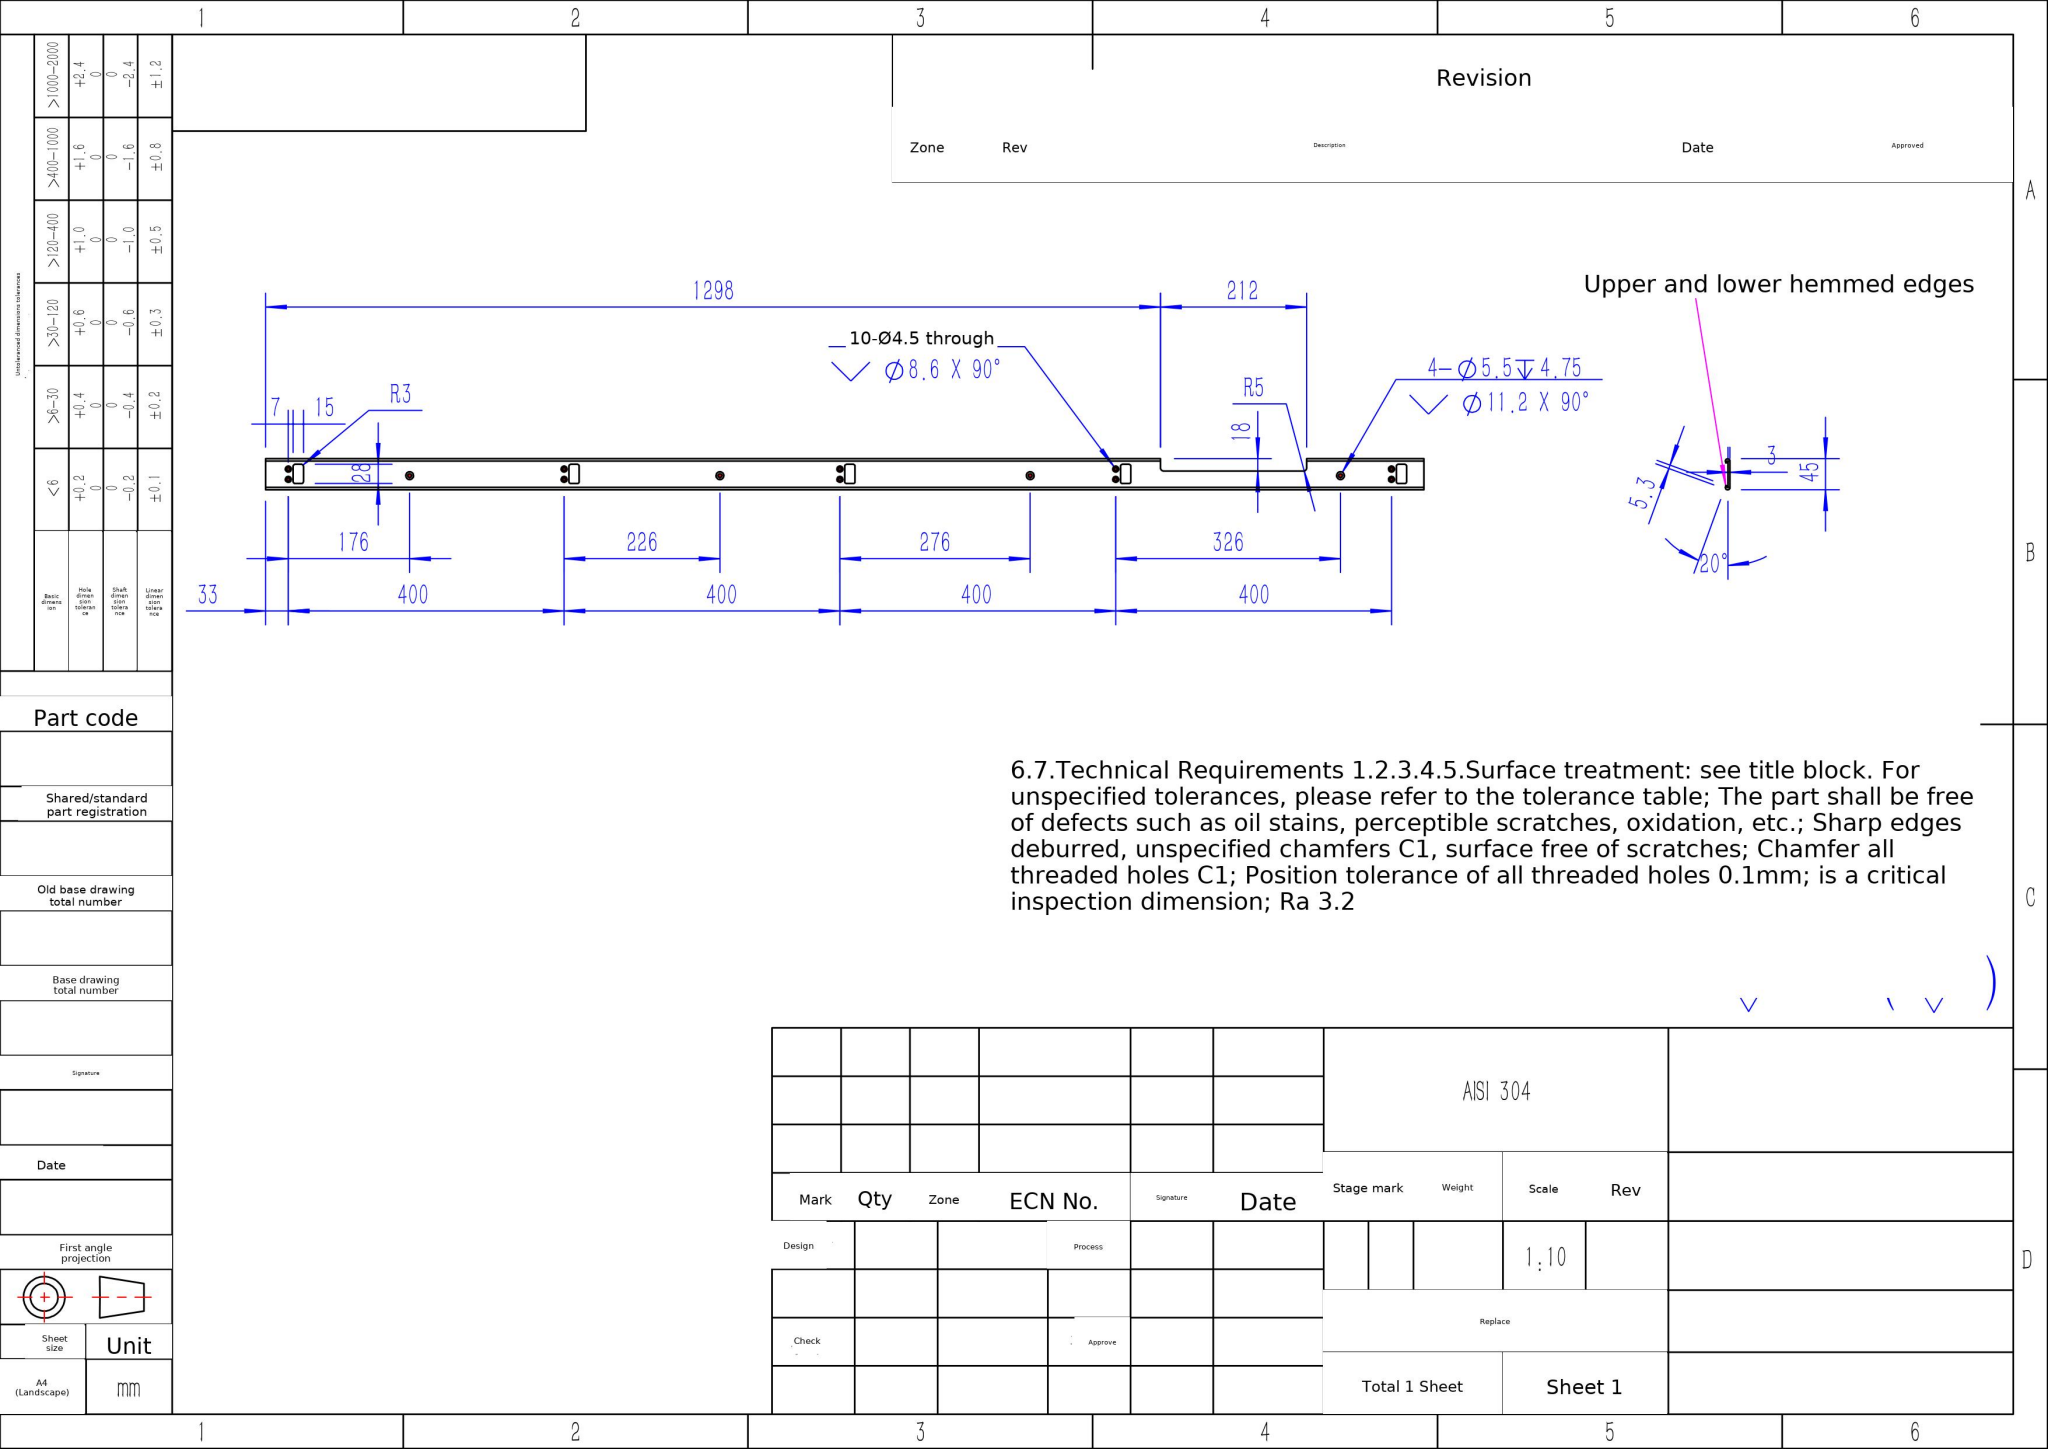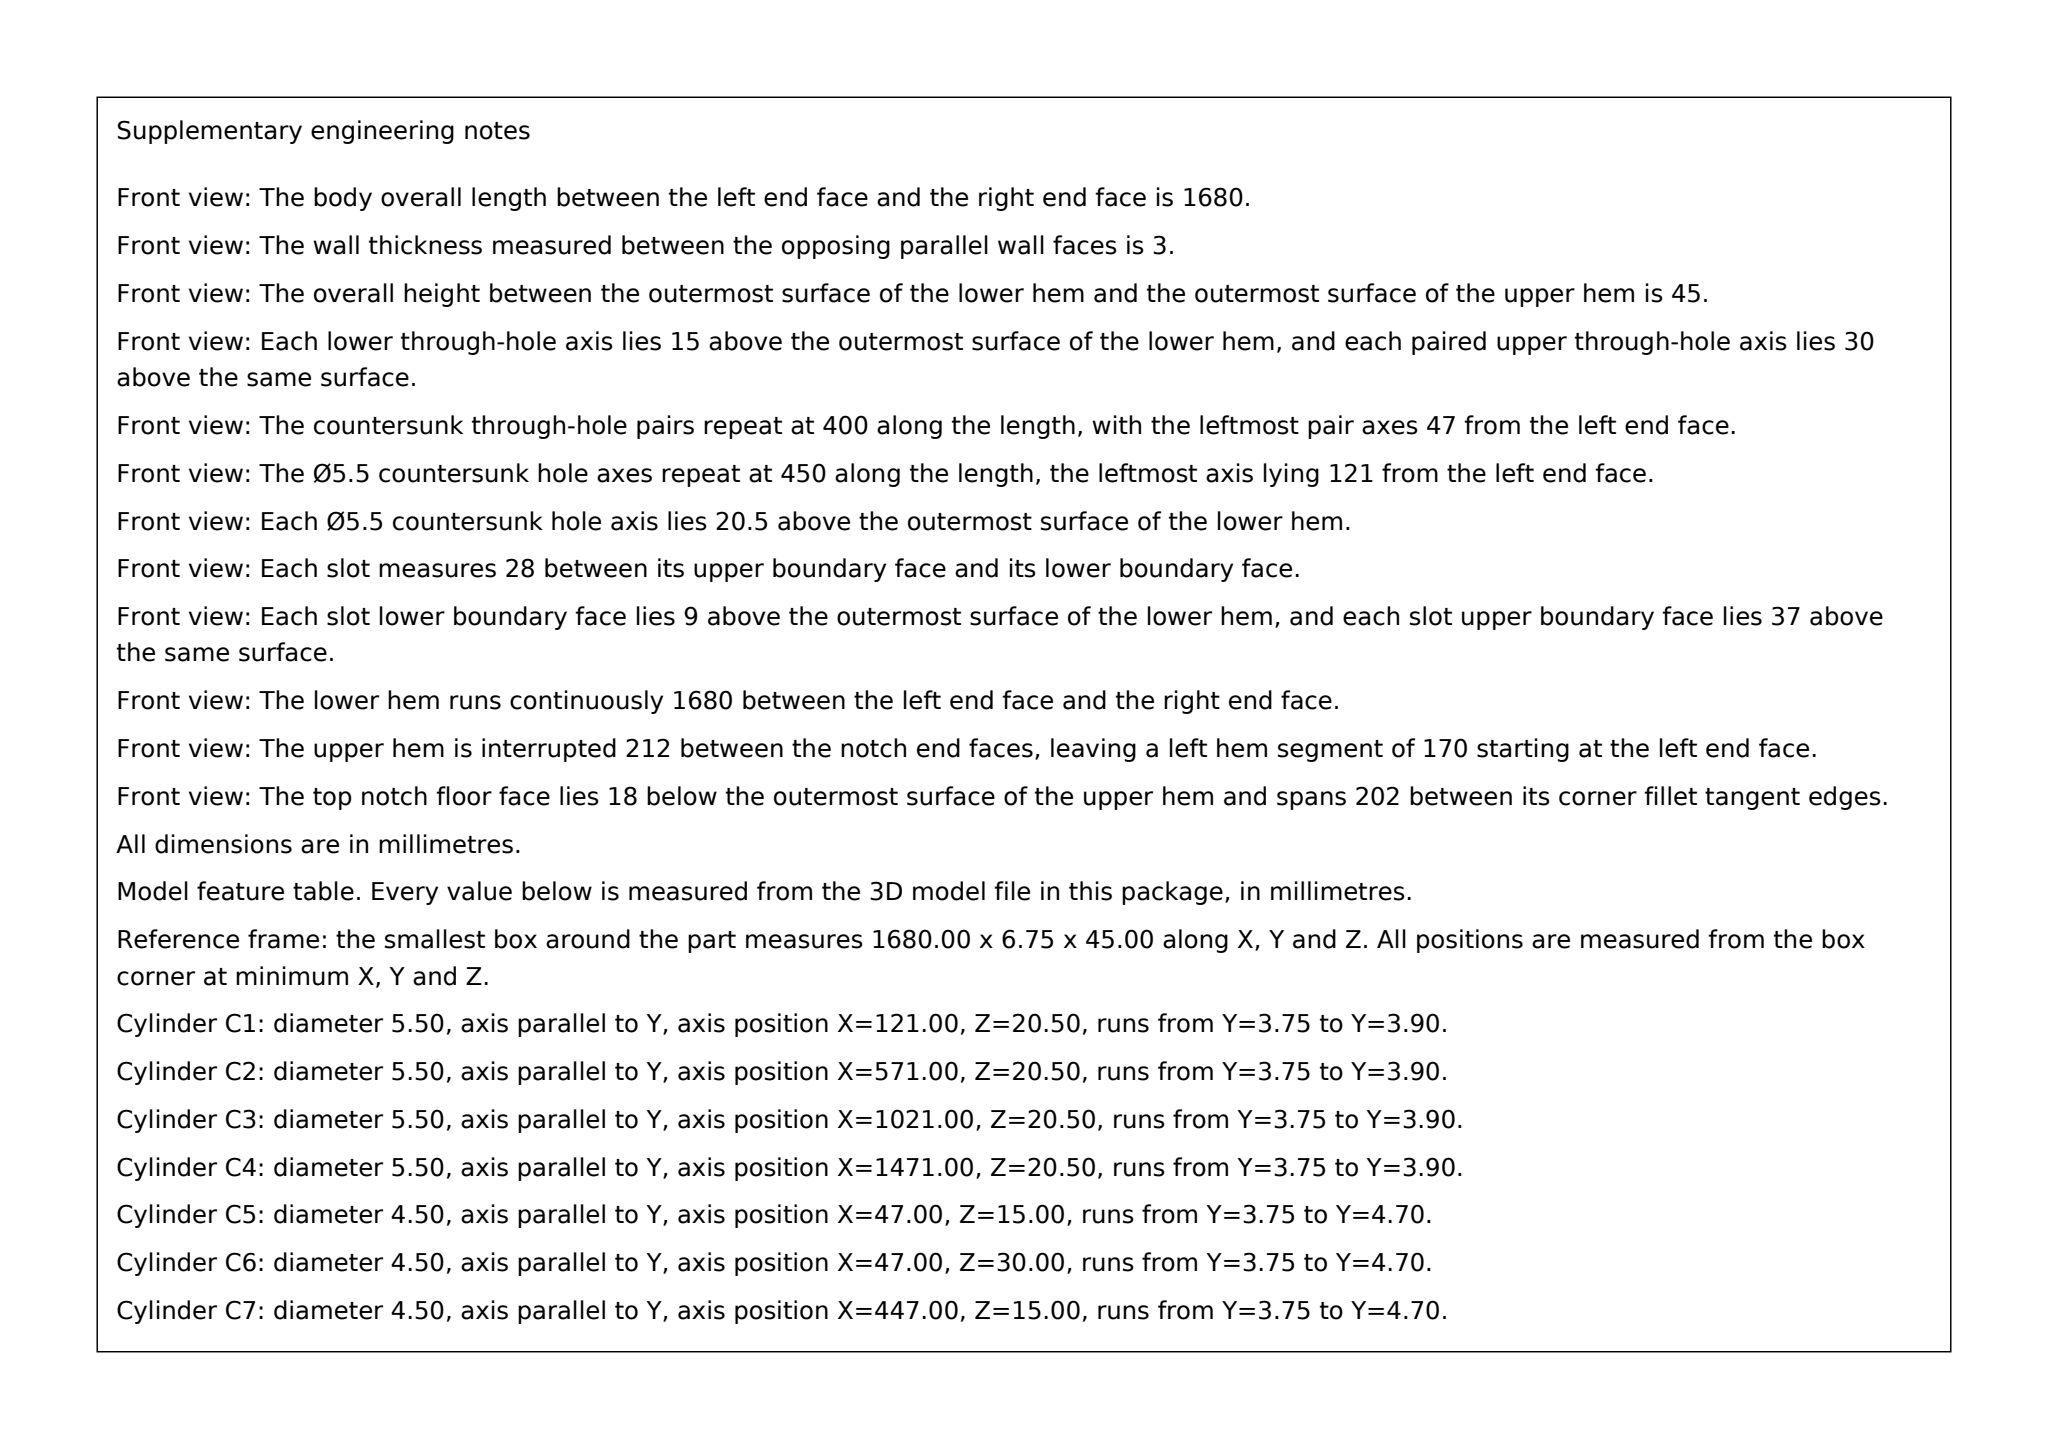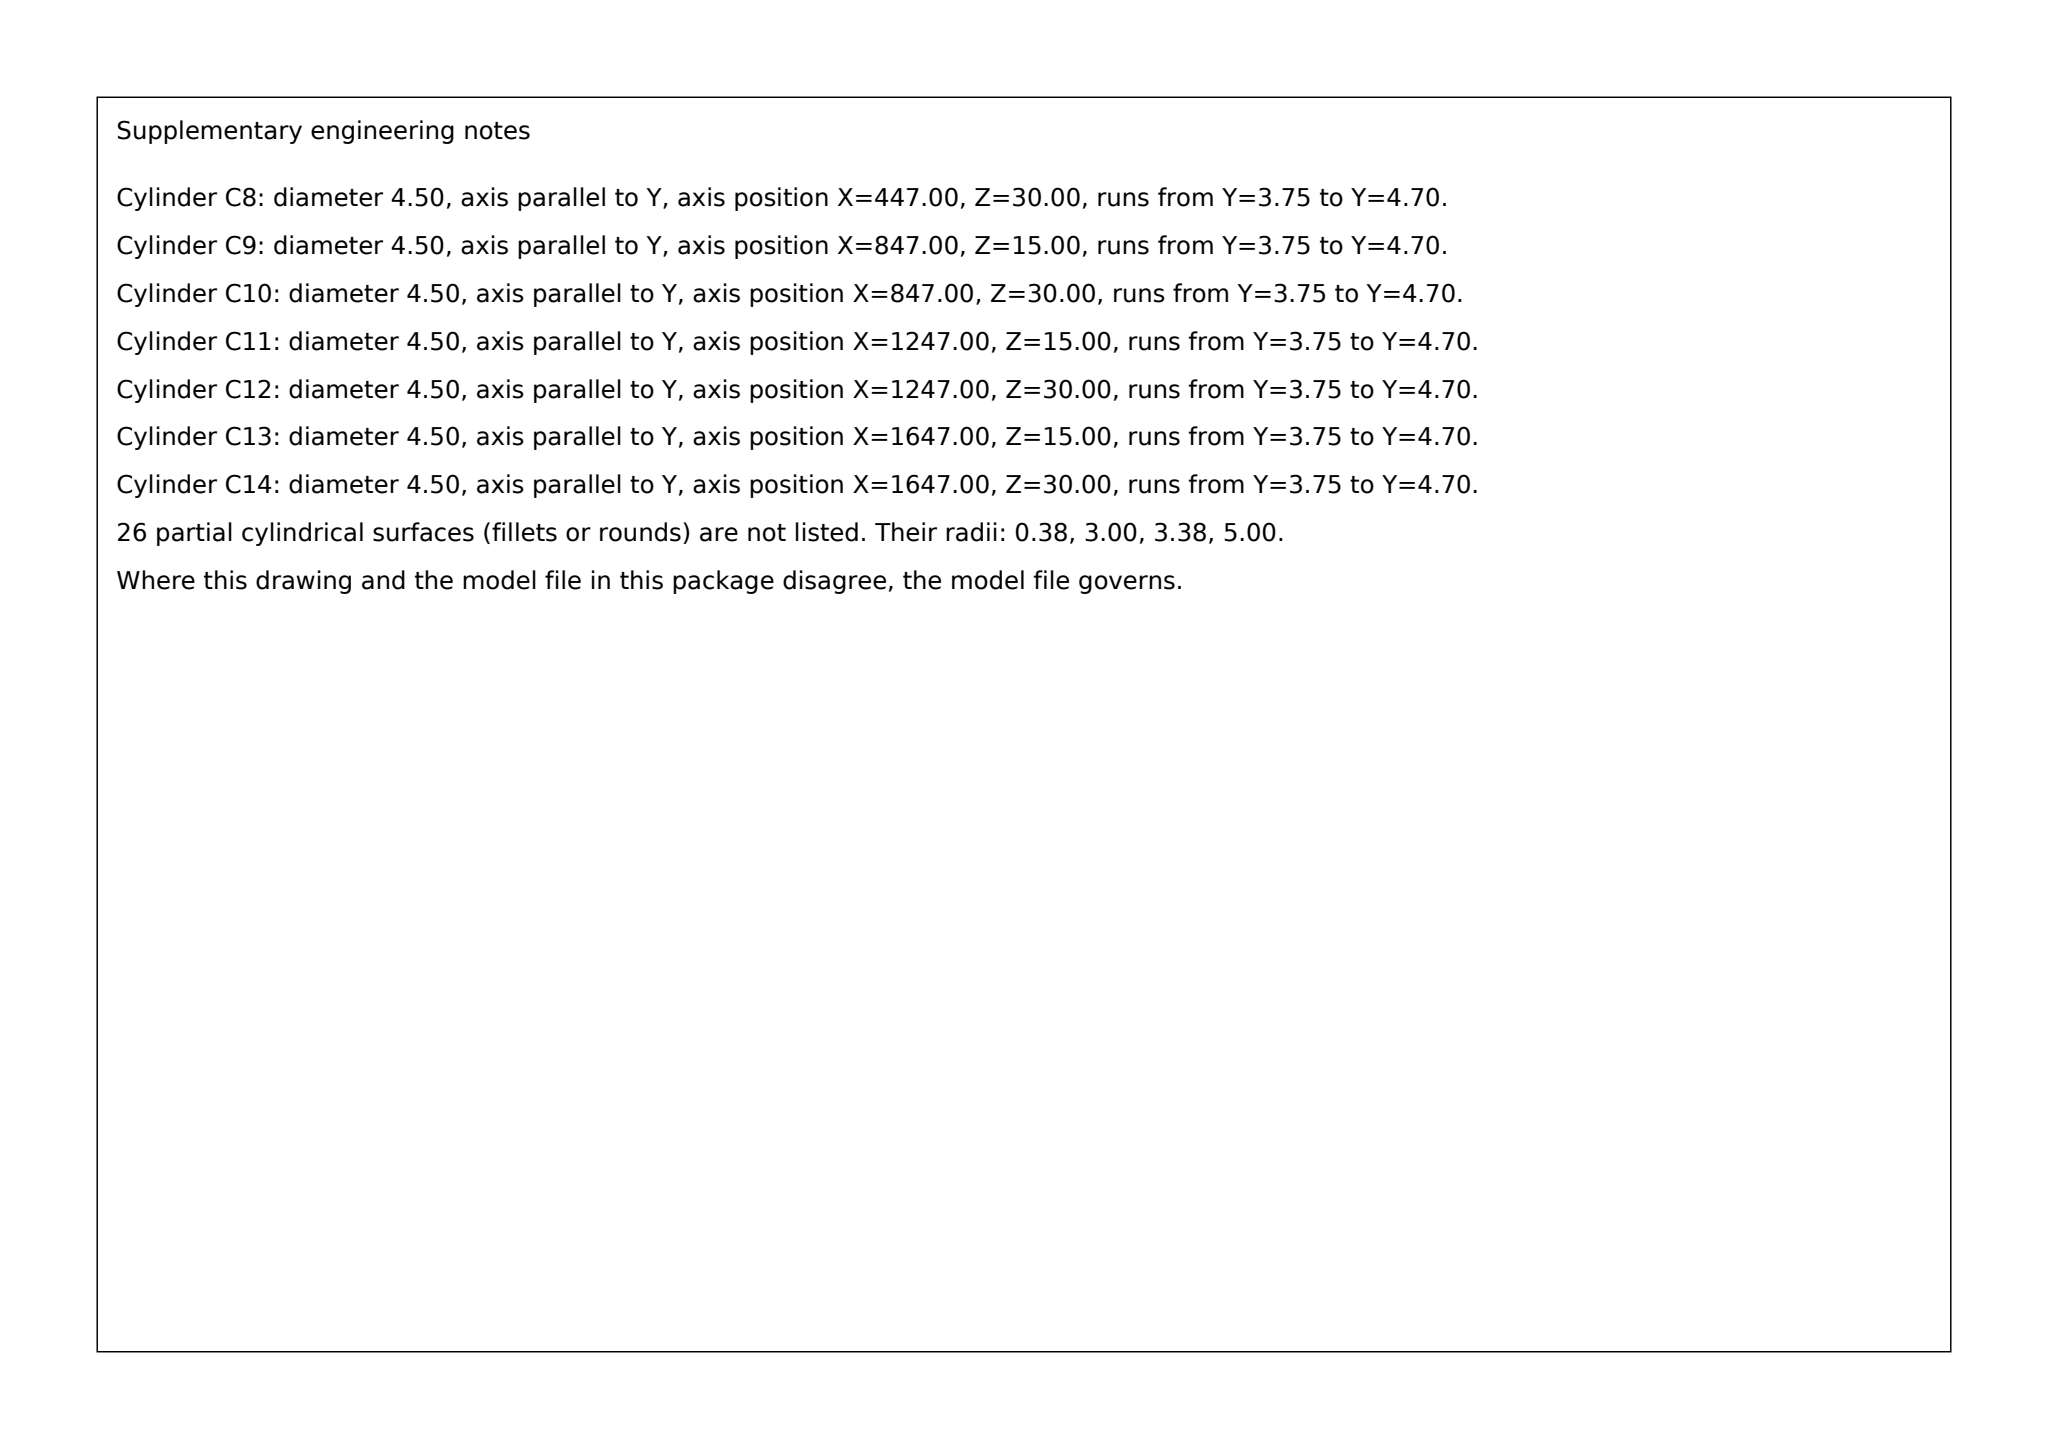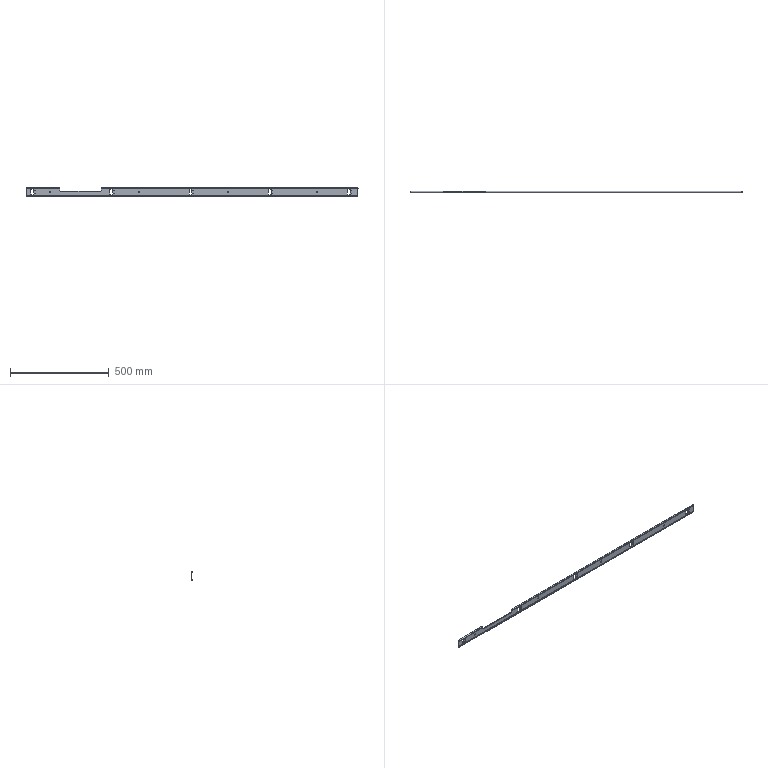Part | SolidWorks | mm | 1 solid | 132 faces | box 1680 x 6.75 x 45 mm | volume 255806 mm3 | cylinder 56 | plane 48 | cone 28 | commonest cylinder face diameters 4.5 x20 6 x20 5.5 x8 6.75 x3 0.75 x3 10 x2
Drawing notes:
5X 15 X 28 CUTOUT: 9 FROM BOTTOM EDGE, 8 FROM TOP EDGE | from the solid: z-planes at 9.0 (x5) and 37.0 (x5); part height 45 -> 9 bottom / 8 top
HEM DETAIL: OPEN GAP 0.75, INSIDE R0.38, FOLDED THK 6.75 | from the solid: bbox Y=6.75; y-planes 3.75 & 6.75 (3 thk skin); R0.375 bend cyl dia 0.75 at y=3.38